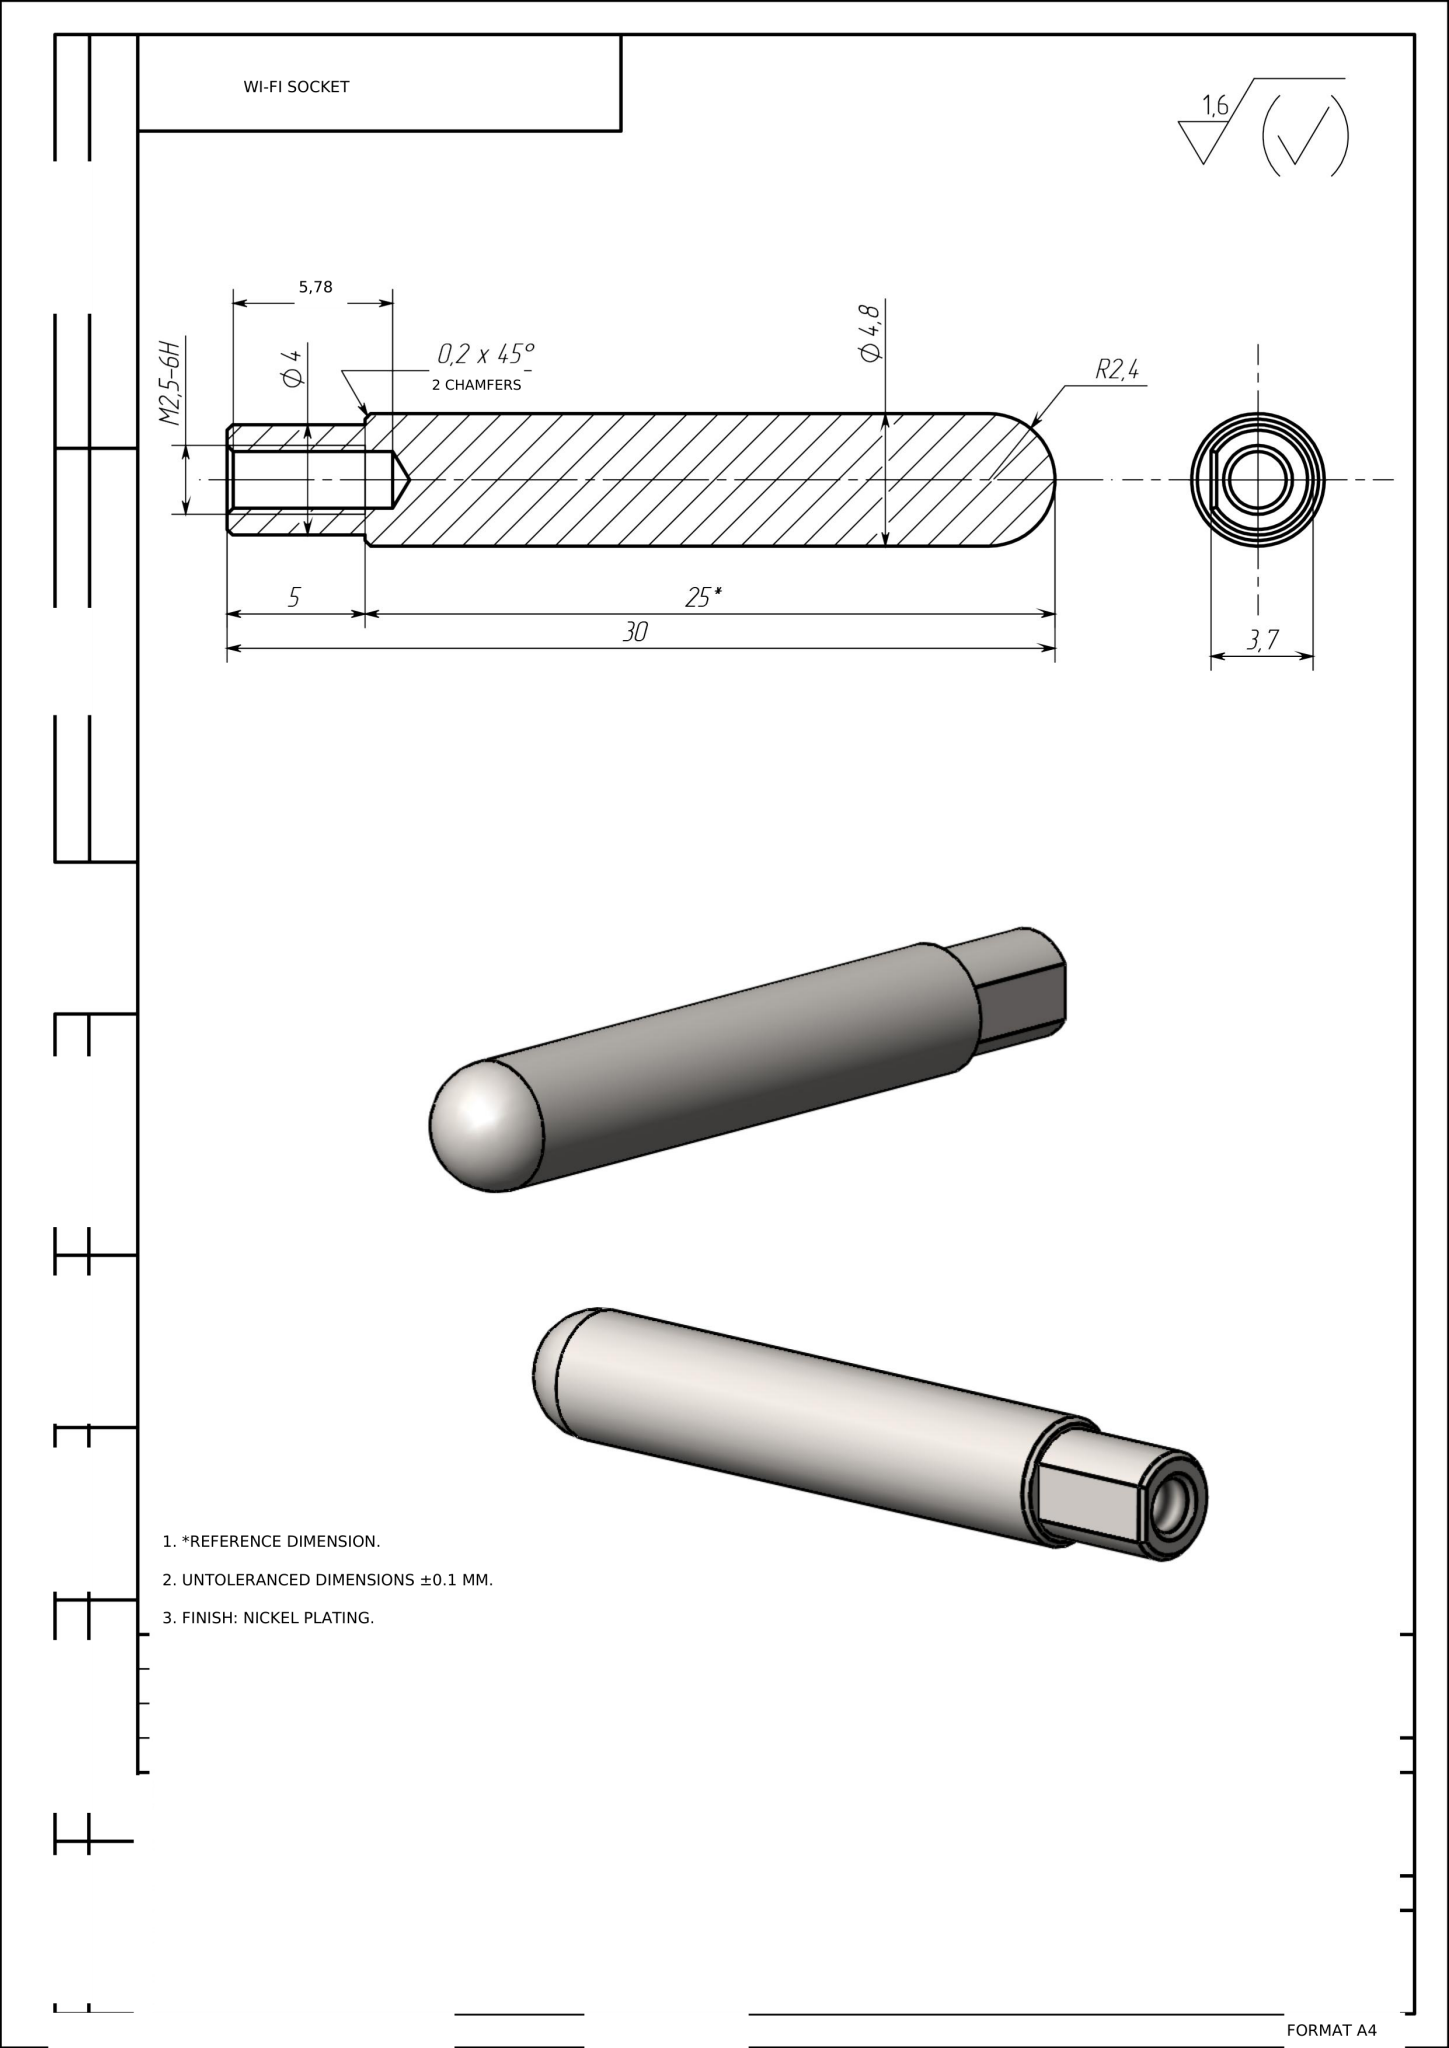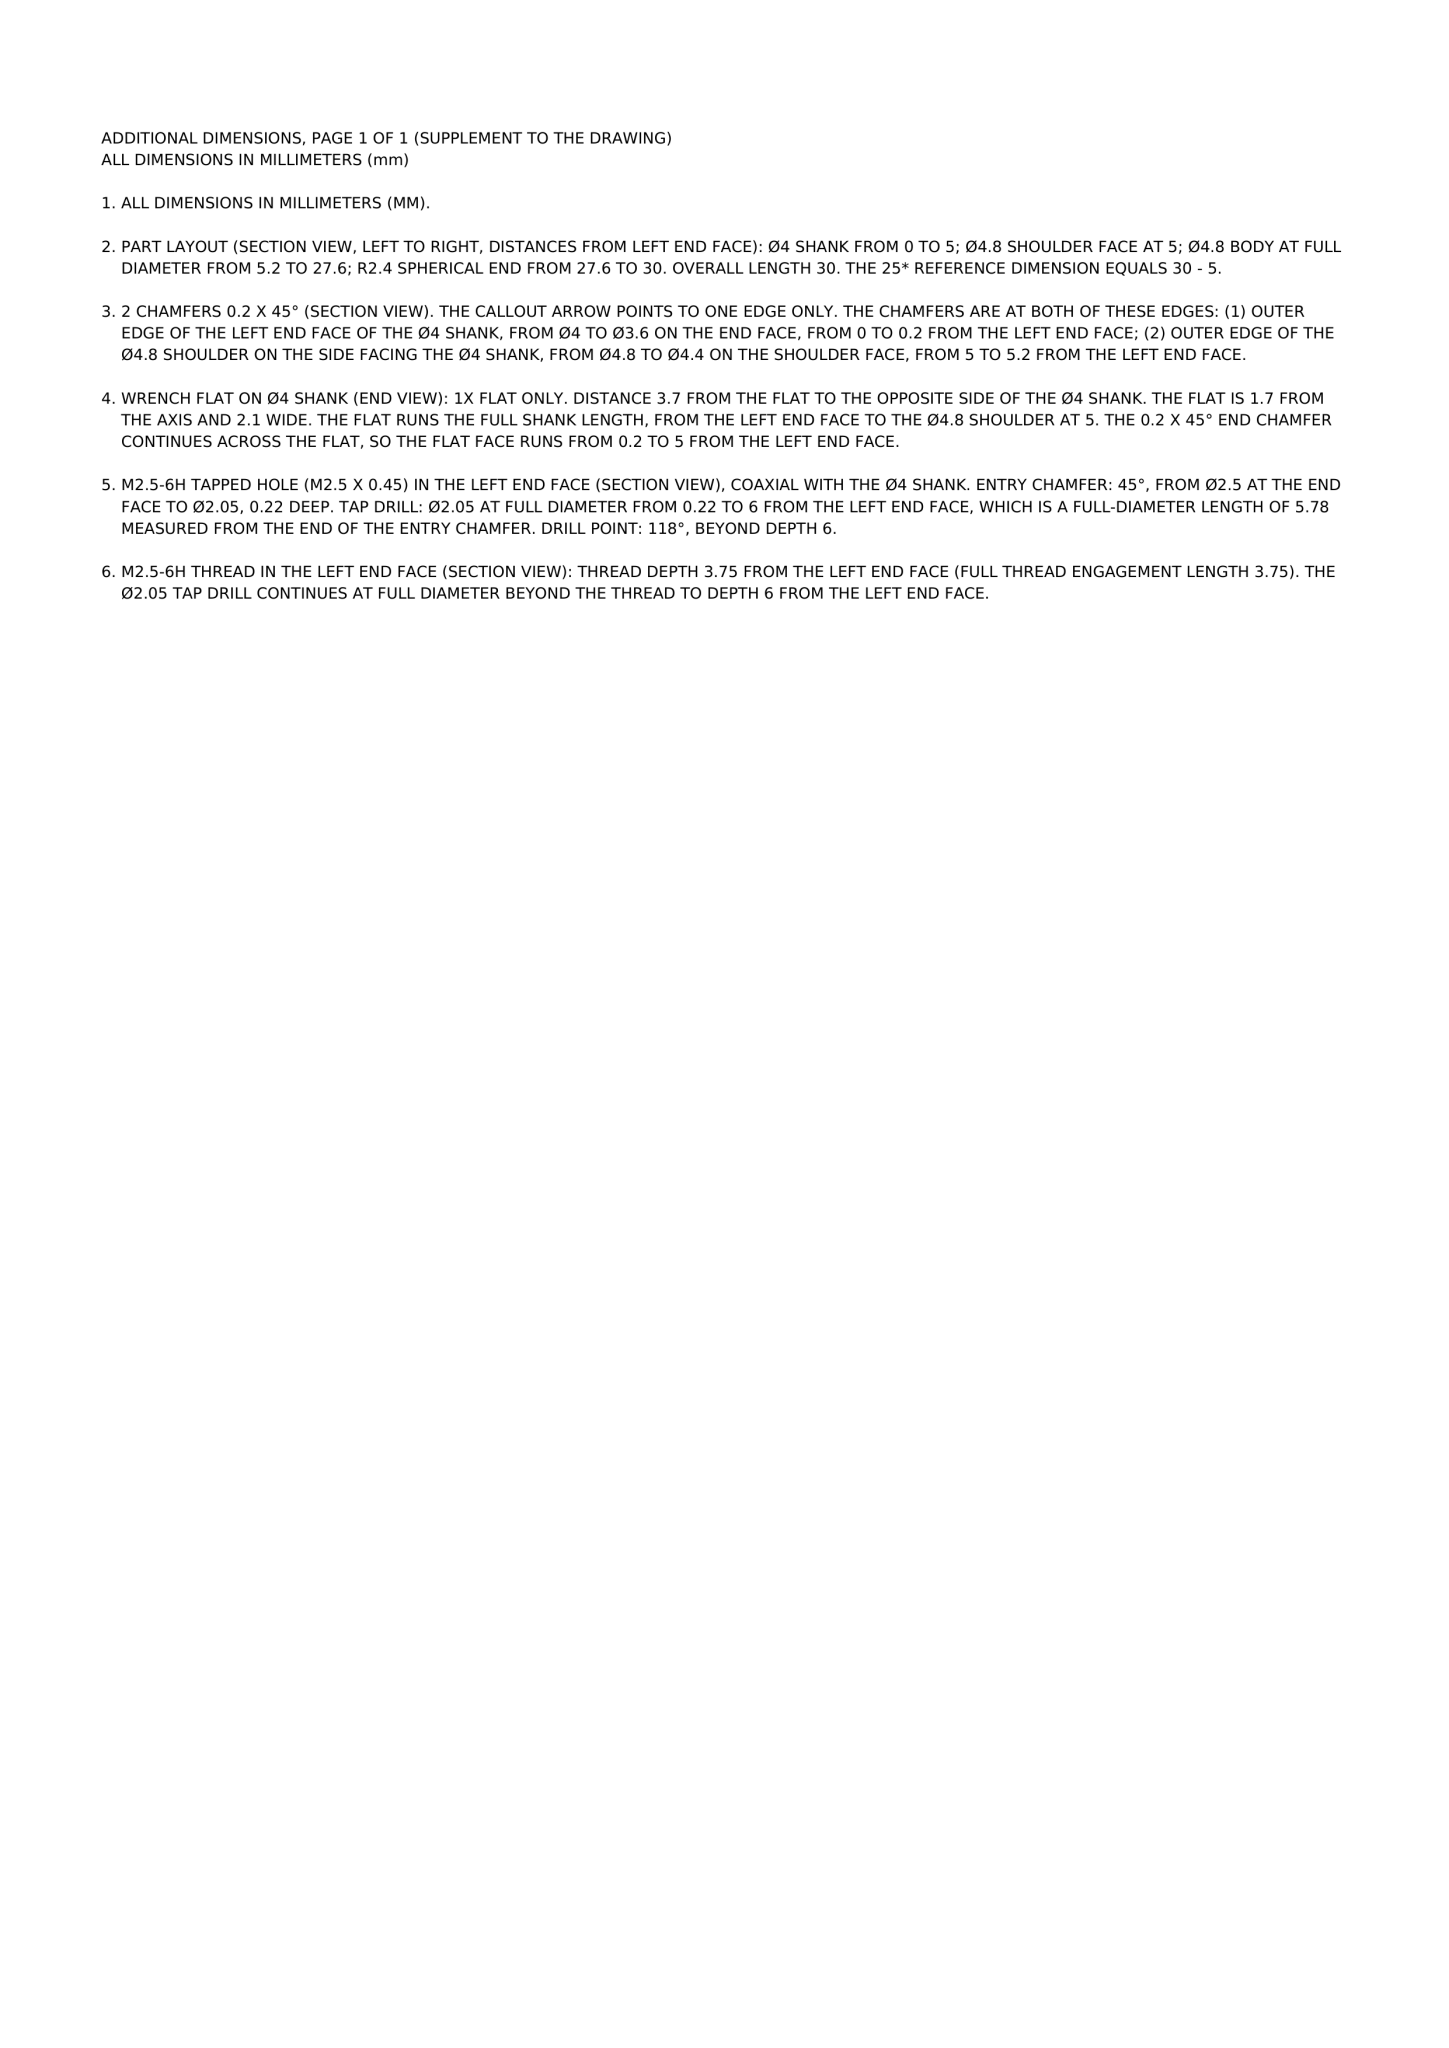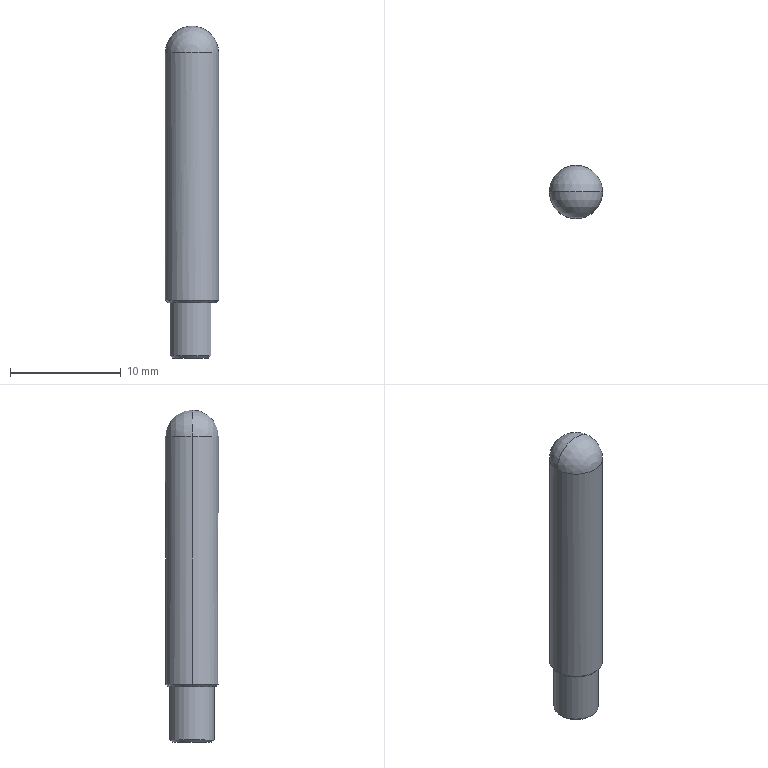Part | NX | mm | 1 solid | 18 faces | box 4.8 x 4.8 x 30 mm | volume 477 mm3 | cone 7 | cylinder 5 | plane 4 | sphere 2 | commonest cylinder face diameters 2.05 x2 4.8 x2 4 x1